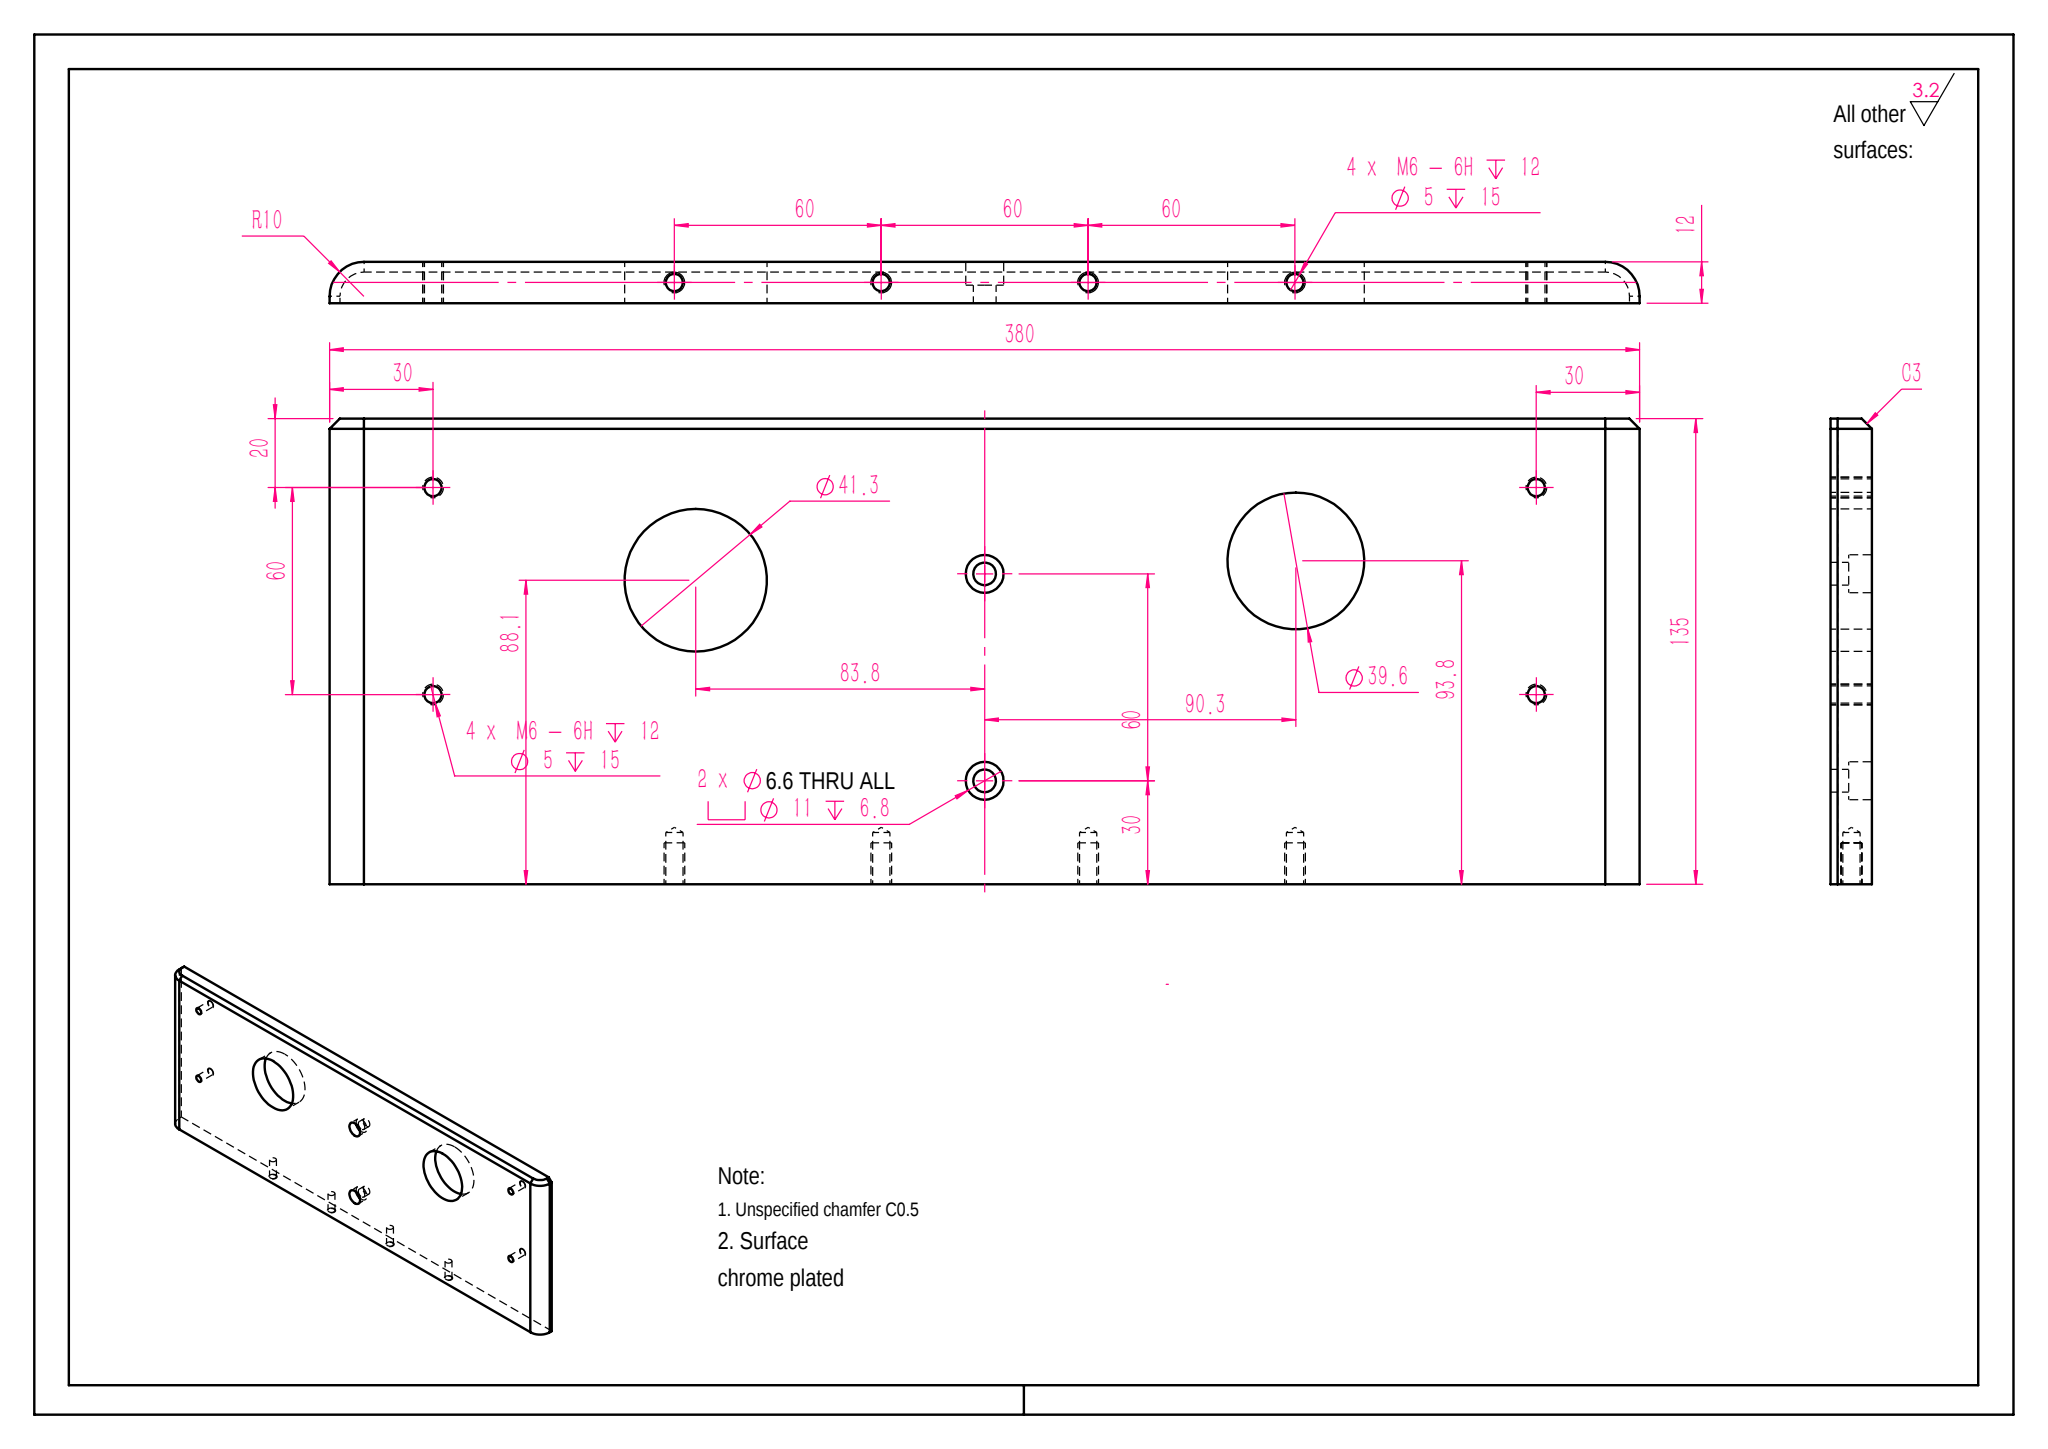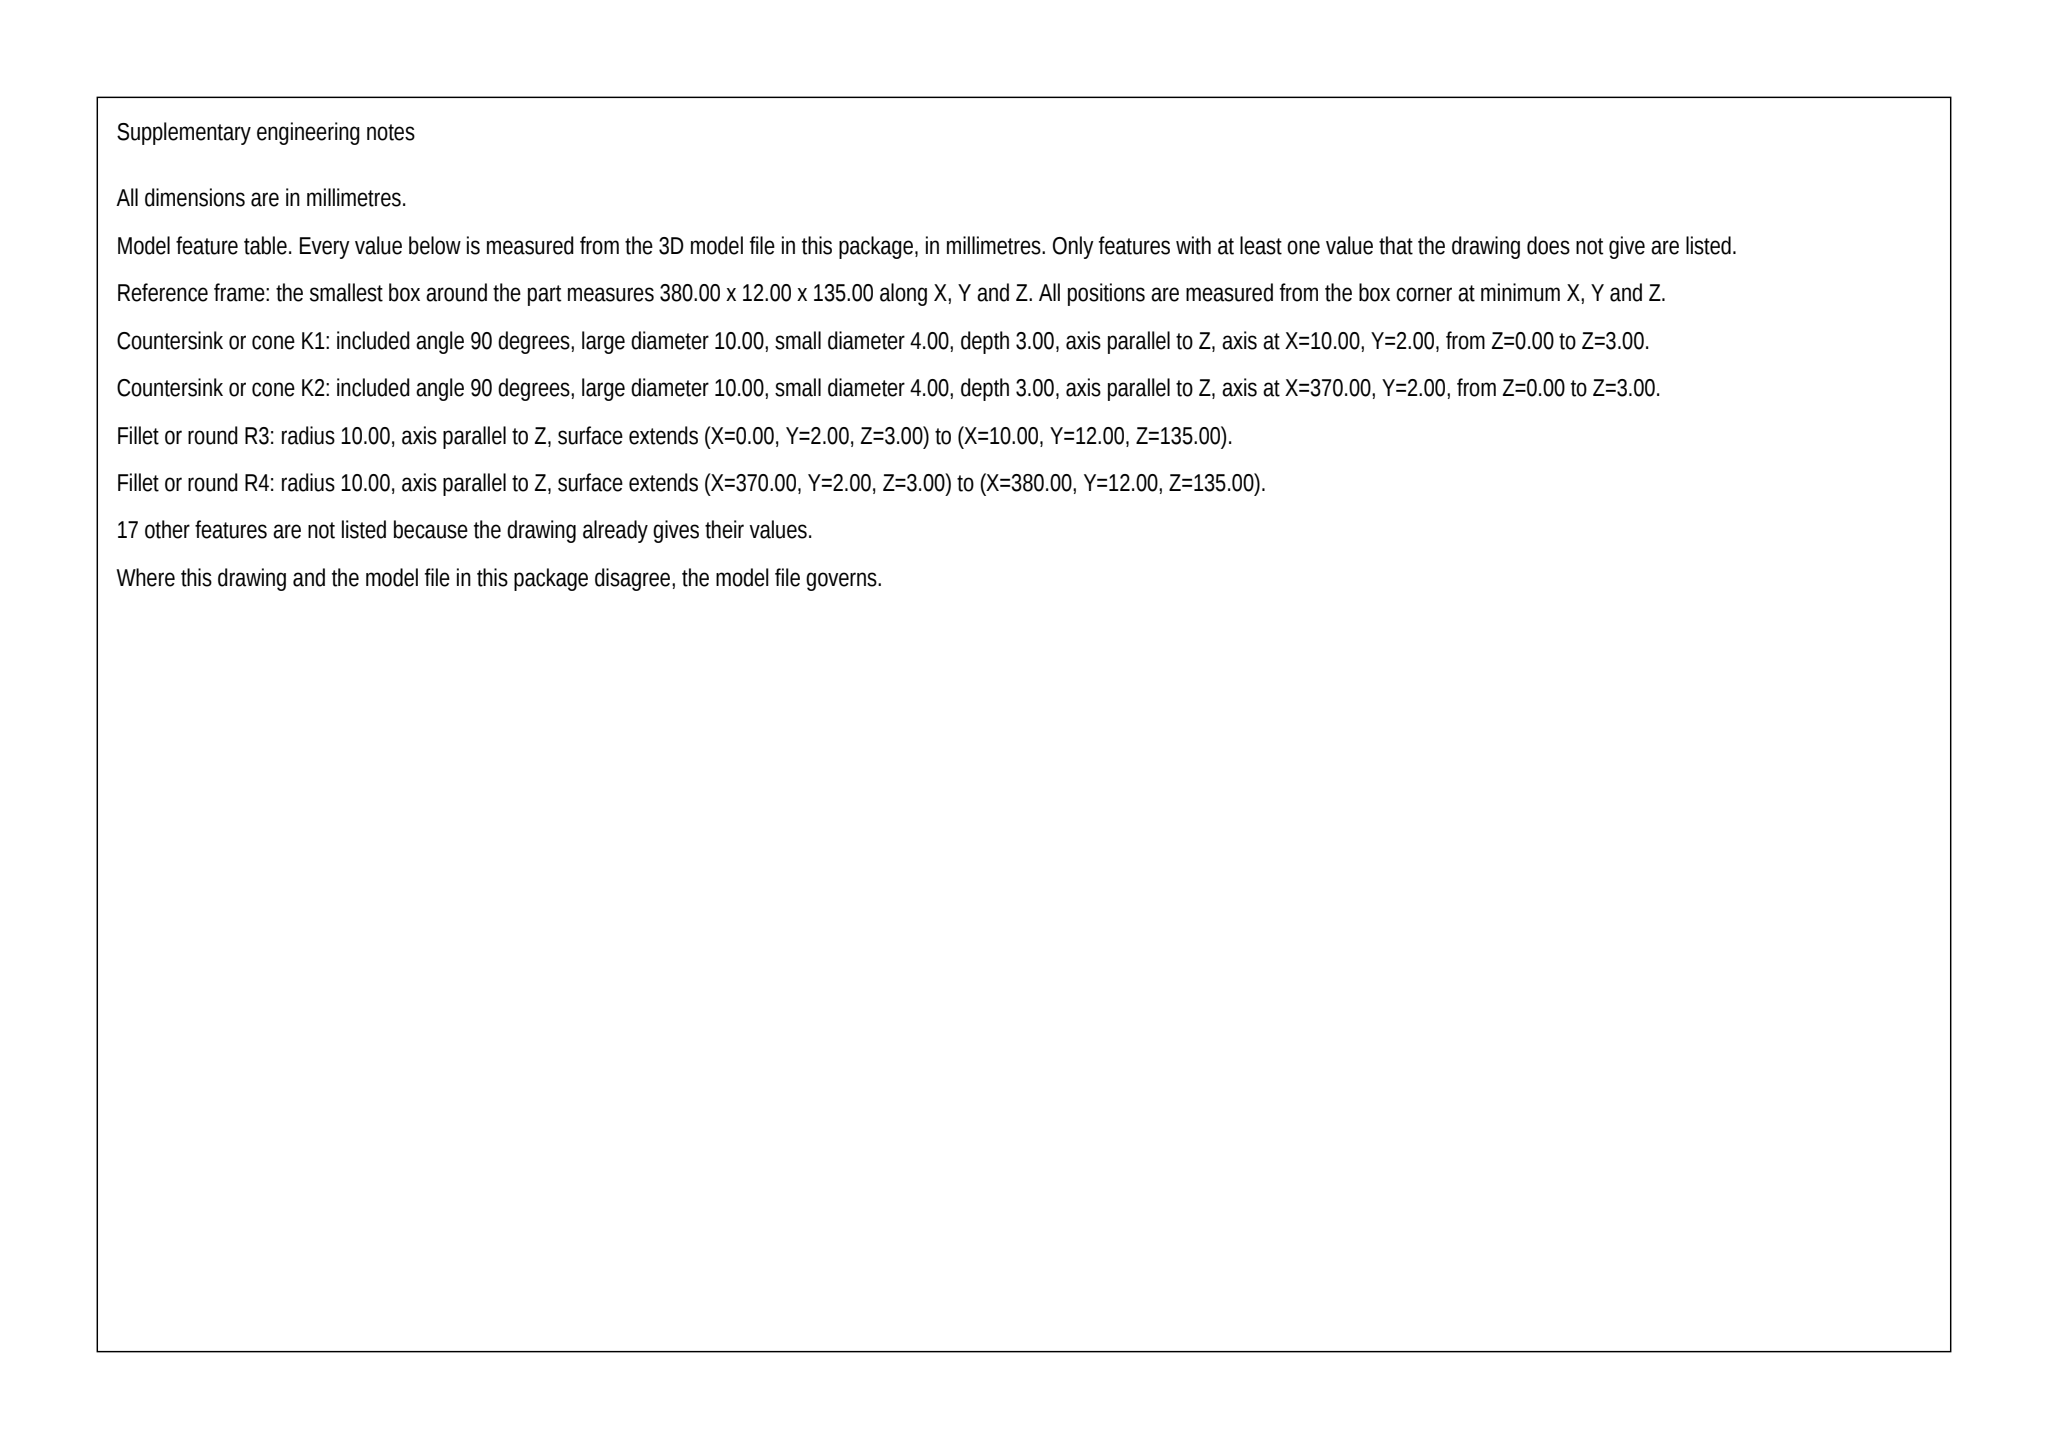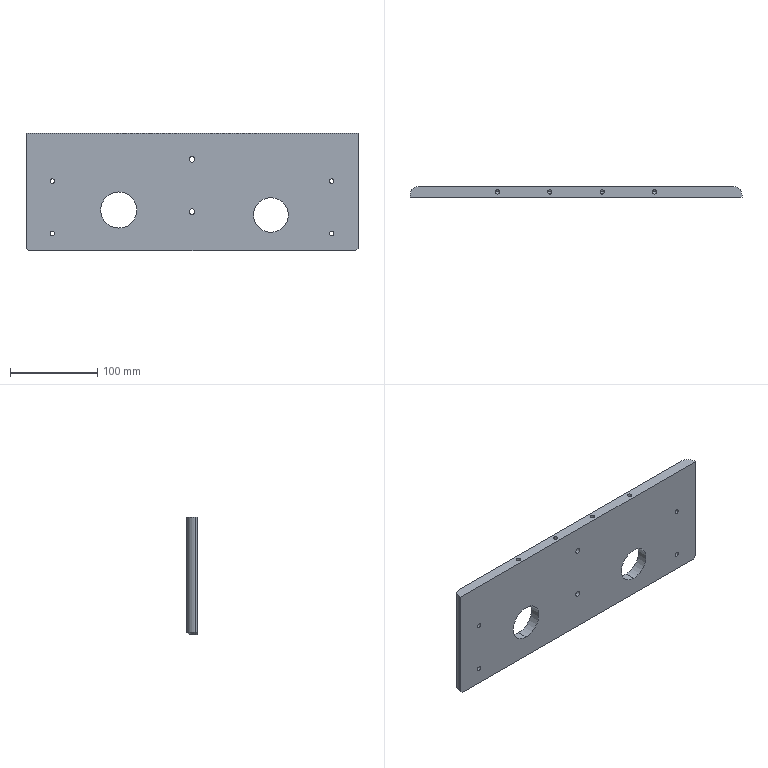Part | SolidWorks | mm | 1 solid | 51 faces | box 380 x 12 x 135 mm | volume 573355 mm3 | cylinder 30 | plane 11 | cone 10 | commonest cylinder face diameters 5 x16 11 x4 6.6 x4 39.639 x2 41.291 x2 20 x2
build123d program:
from build123d import *

# Parameters (mm, degrees)
SKETCH1_W                                            = 380
SKETCH1_H                                            = 135
BOSS_EXTRUDE1_DEPTH                                  = 12
M6_TAPPED_HOLE2_D                                    = 5
M6_TAPPED_HOLE2_DEPTH                                = 15
M6_TAPPED_HOLE2_TIP                                  = 1.502
FILLET1_R                                            = 10
CHAMFER1_SIZE                                        = 3
M6_TAPPED_HOLE1_D                                    = 5
M6_TAPPED_HOLE1_DEPTH                                = 15
M6_TAPPED_HOLE1_TIP                                  = 1.502
HOLE_SIZE_ACCORDING_TO_HEXAGON_SOCKET_HE_D           = 6.6
HOLE_SIZE_ACCORDING_TO_HEXAGON_SOCKET_HE_CBORE_D     = 11
HOLE_SIZE_ACCORDING_TO_HEXAGON_SOCKET_HE_CBORE_DEPTH = 6.8
SKETCH8_R                                            = 19.82
SKETCH8_R_2                                          = 20.646
CUT_EXTRUDE1_DEPTH                                   = 80


with BuildPart() as part:
    # Sketch1 → Boss-Extrude1 (new body)
    with BuildSketch(Plane(origin=(0, 0, 0), x_dir=(1, 0, 0), z_dir=(0, 1, 0))):
        Rectangle(SKETCH1_W, SKETCH1_H)
    extrude(amount=BOSS_EXTRUDE1_DEPTH)

    # M6 Tapped Hole2
    with Locations(Plane.XY.offset(67.5)):
        with Locations((-90, 6), (-30, 6), (30, 6), (90, 6)):
            Hole(M6_TAPPED_HOLE2_D / 2, depth=M6_TAPPED_HOLE2_DEPTH)
            with Locations((0, 0, -(M6_TAPPED_HOLE2_DEPTH + M6_TAPPED_HOLE2_TIP / 2))):  # 118° drill point
                Cone(0, M6_TAPPED_HOLE2_D / 2, M6_TAPPED_HOLE2_TIP, mode=Mode.SUBTRACT)

    # Fillet1
    fillet1_edges = [part.edges().sort_by_distance(p)[0] for p in [
        (-190, 12, 0),
        (190, 12, 0),
    ]]
    fillet(fillet1_edges, radius=FILLET1_R)

    # Chamfer1
    chamfer1_edges = [part.edges().sort_by_distance(p)[0] for p in [
        (0, 12, -67.5),
        (-190, 1, -67.5),
        (190, 1, -67.5),
        (-187.071, 9.071, -67.5),
        (187.071, 9.071, -67.5),
    ]]
    chamfer(chamfer1_edges, length=CHAMFER1_SIZE)

    # M6 Tapped Hole1
    with Locations(Plane(origin=(0, 0, 0), x_dir=(-1, 0, 0), z_dir=(0, -1, 0))):
        with Locations((160, -12.5), (160, 47.5), (-160, -12.5), (-160, 47.5)):
            Hole(M6_TAPPED_HOLE1_D / 2, depth=M6_TAPPED_HOLE1_DEPTH)
            with Locations((0, 0, -(M6_TAPPED_HOLE1_DEPTH + M6_TAPPED_HOLE1_TIP / 2))):  # 118° drill point
                Cone(0, M6_TAPPED_HOLE1_D / 2, M6_TAPPED_HOLE1_TIP, mode=Mode.SUBTRACT)

    # Hole Size according to Hexagon Socket He (through all)
    with Locations(Plane(origin=(0, 12, 0), x_dir=(1, 0, 0), z_dir=(0, 1, 0))):
        with Locations((0, -37.5), (0, 22.5)):
            CounterBoreHole(HOLE_SIZE_ACCORDING_TO_HEXAGON_SOCKET_HE_D / 2, HOLE_SIZE_ACCORDING_TO_HEXAGON_SOCKET_HE_CBORE_D / 2, HOLE_SIZE_ACCORDING_TO_HEXAGON_SOCKET_HE_CBORE_DEPTH)

    # Sketch8 → Cut-Extrude1 (cut)
    with BuildSketch(Plane(origin=(0, 0, 0), x_dir=(-1, 0, 0), z_dir=(0, -1, 0))):
        with Locations(Location((-90.264, 26.26, 0), (0, 0, 90))):
            Circle(SKETCH8_R)
        with Locations(Location((83.786, 20.646, 0), (0, 0, 90))):
            Circle(SKETCH8_R_2)
    extrude(amount=-CUT_EXTRUDE1_DEPTH, mode=Mode.SUBTRACT)


solid = part.part